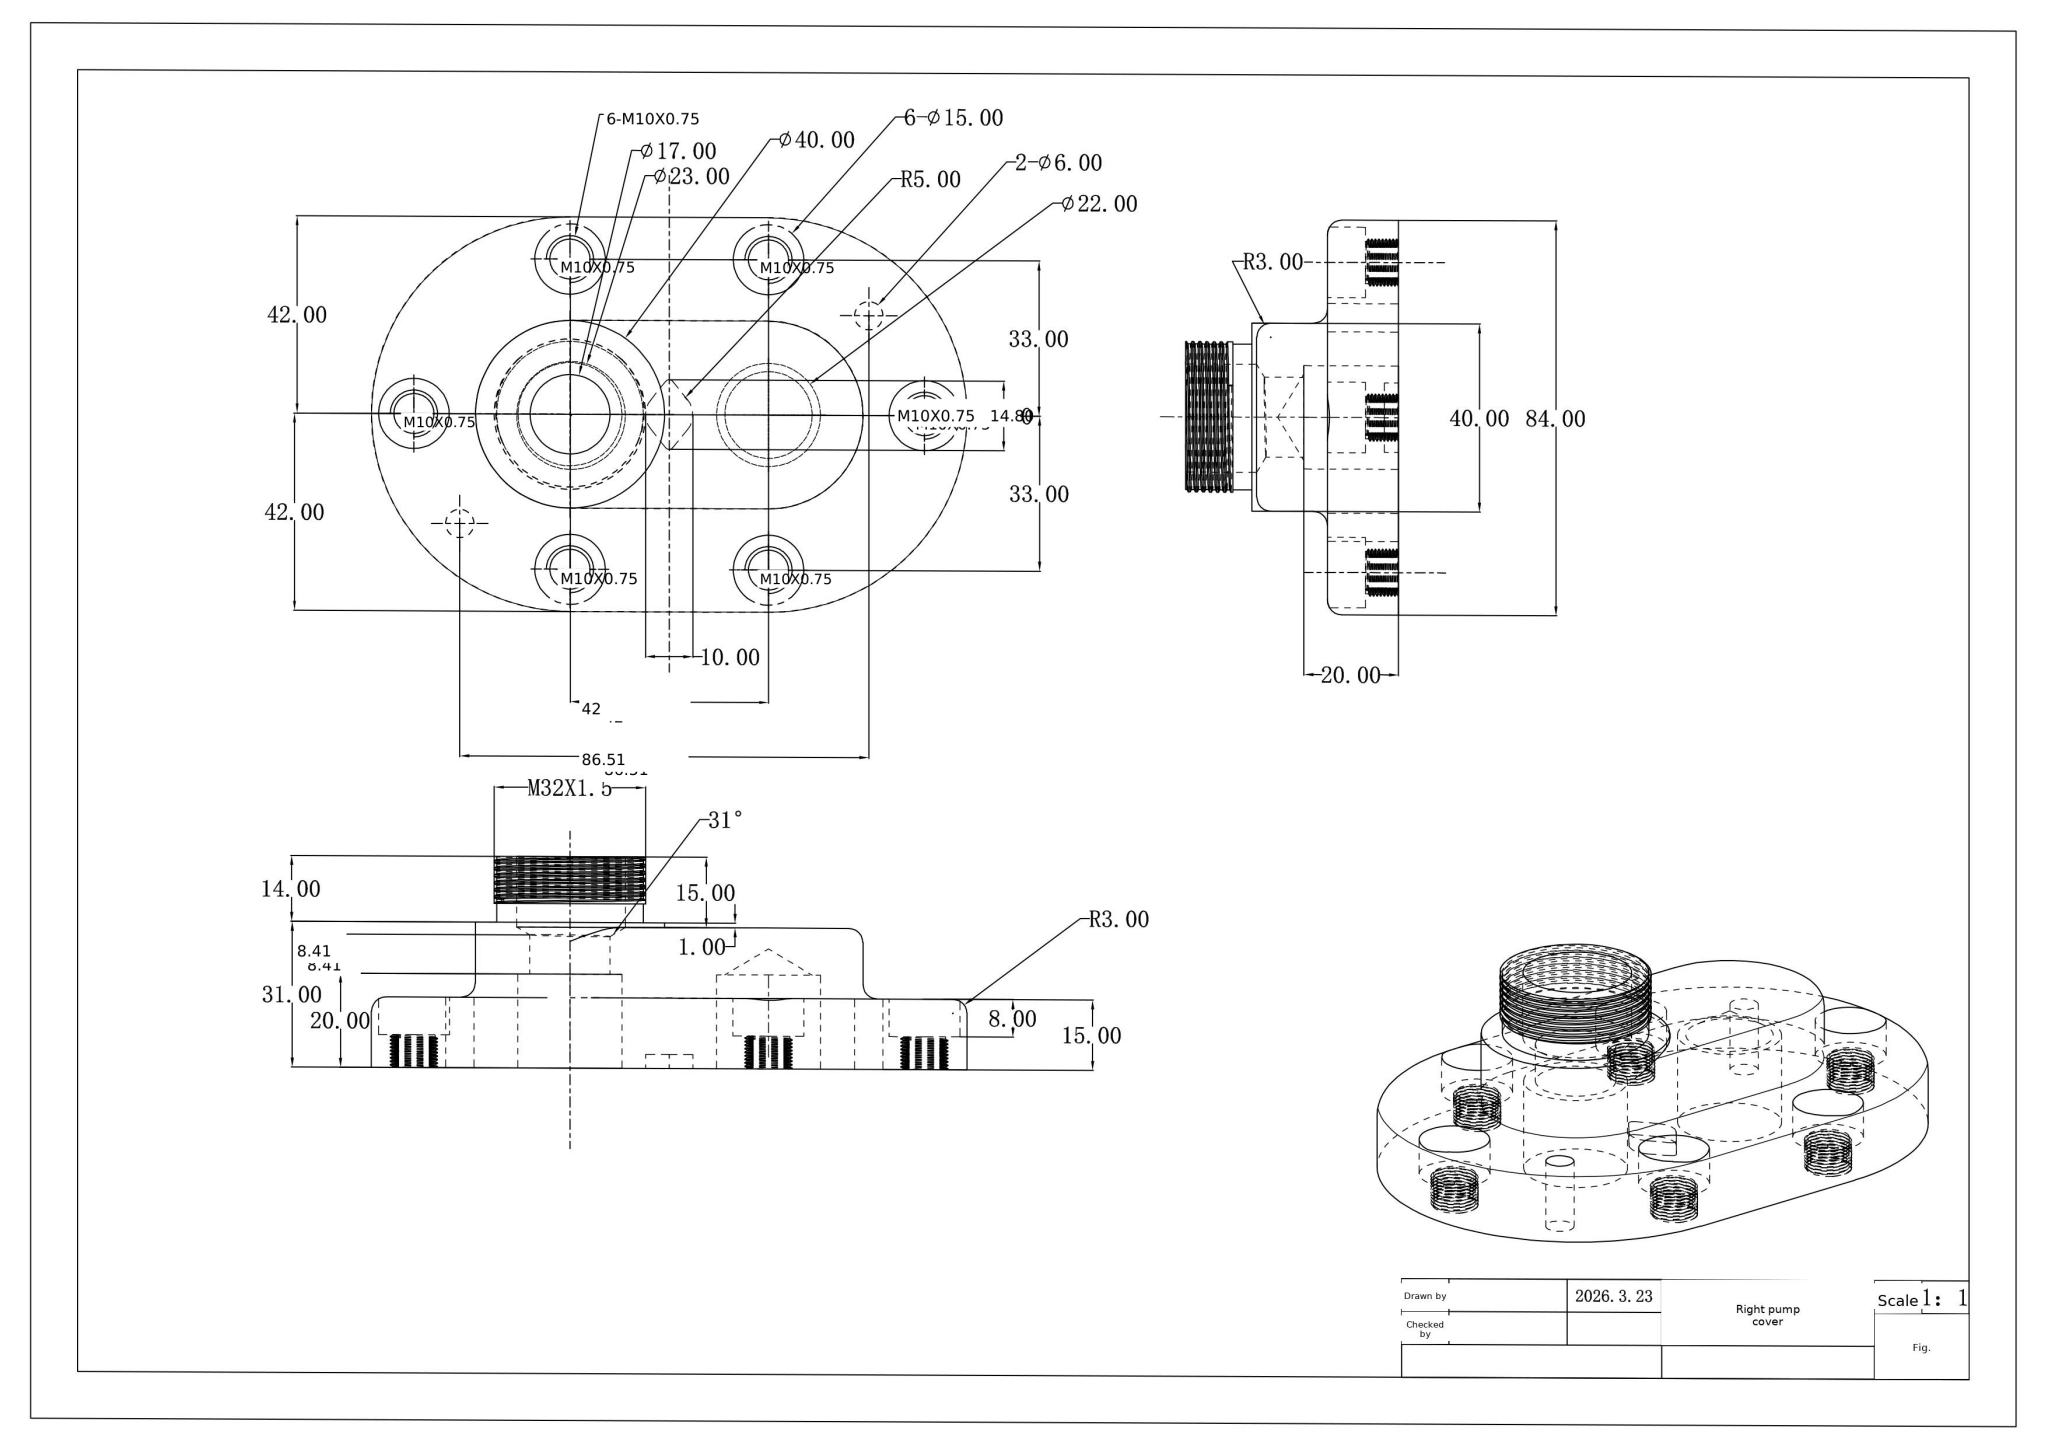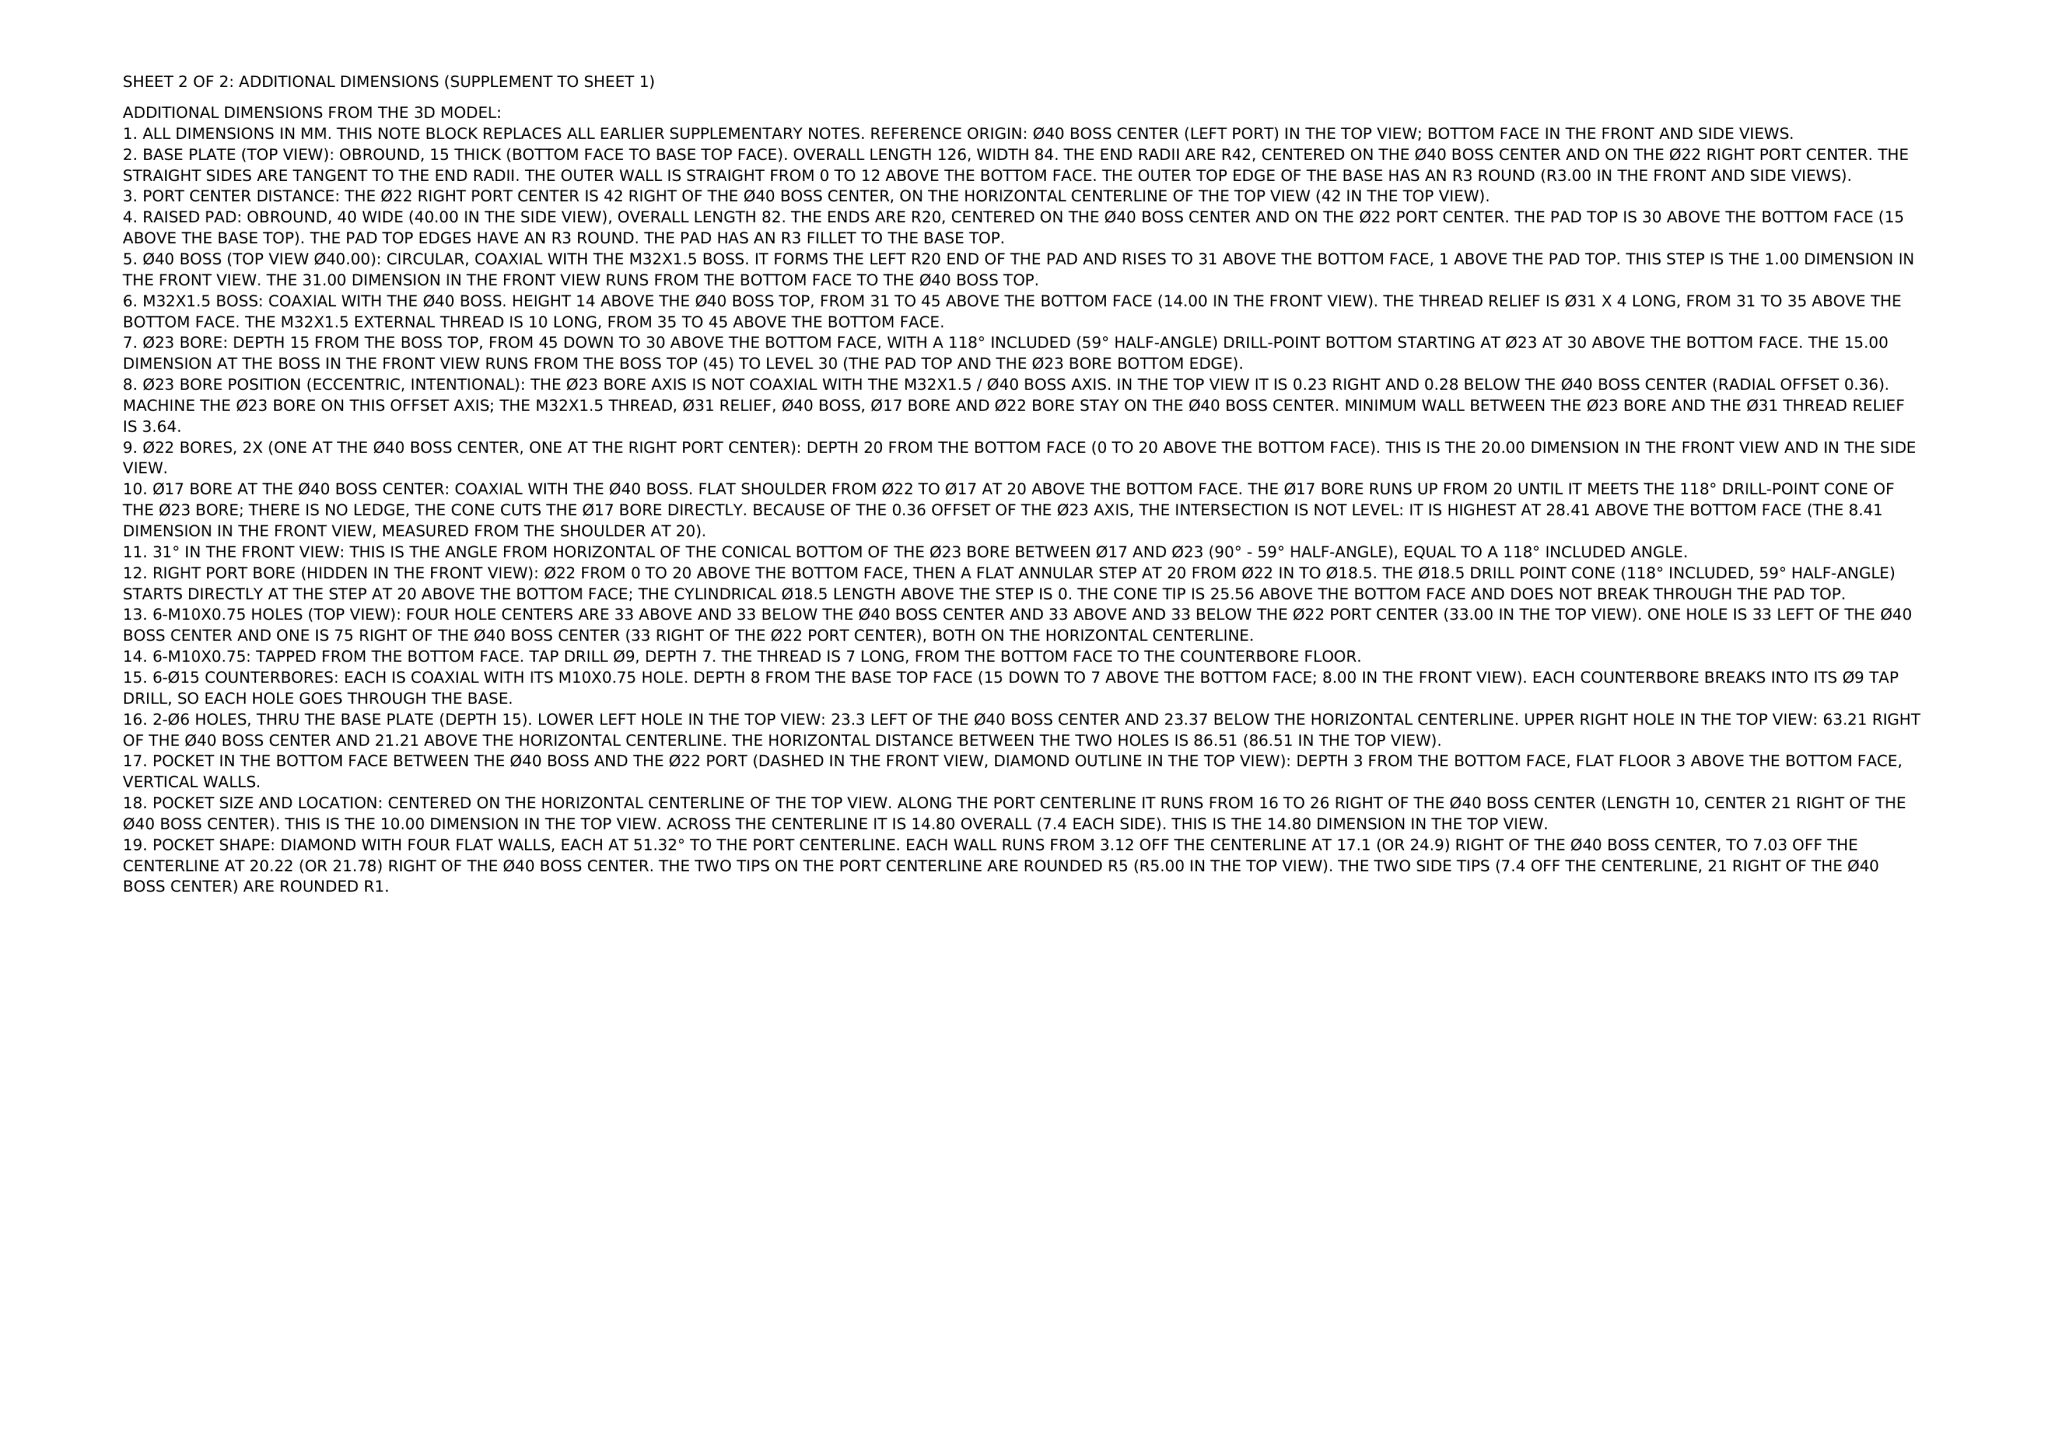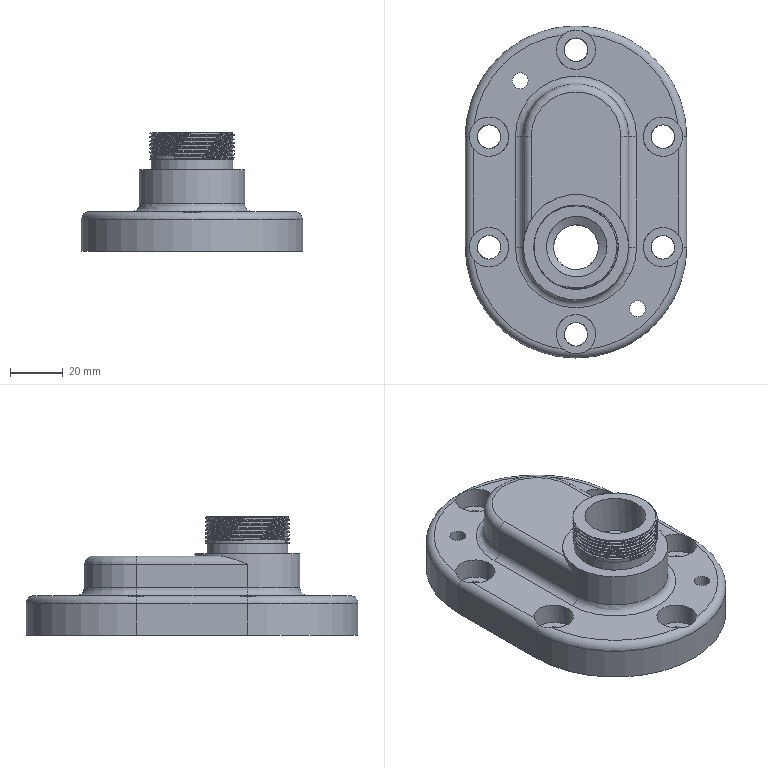Part | NX | mm | 1 solid | 92 faces | box 84 x 126 x 45 mm | volume 154677 mm3 | cylinder 41 | plane 30 | spline 14 | torus 5 | cone 2 | commonest cylinder face diameters 6 x8 10 x8 9 x6 15 x6 84 x2 40 x2 31 x2 22 x2